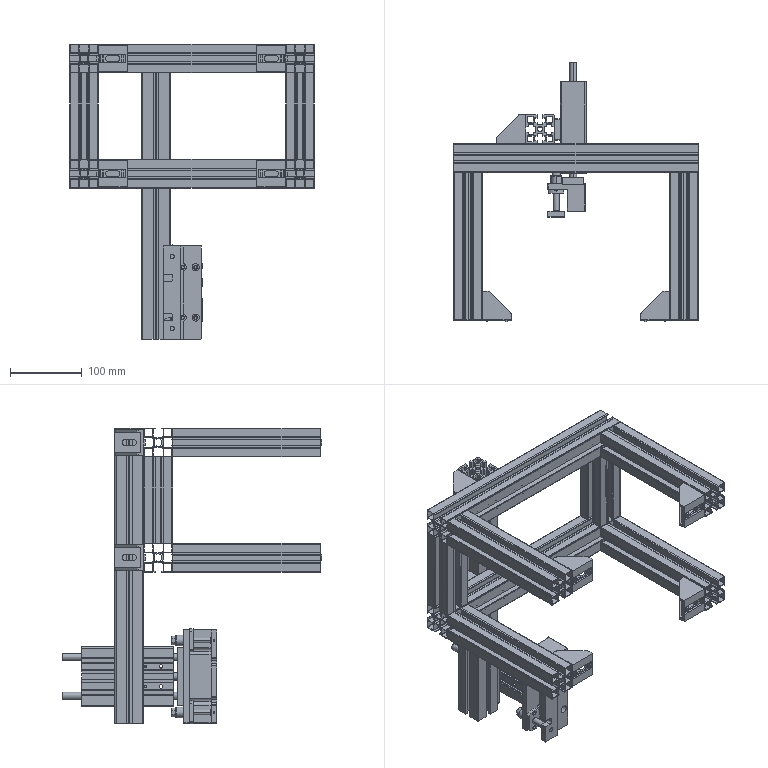Assembly | SolidWorks | mm | 17 component files | 24 solids | 1667 faces | box 340 x 360.1 x 411 mm | volume 1426037 mm3 | plane 1046 | cylinder 493 | cone 122 | spline 6 | commonest cylinder face diameters 4 x64 2.8 x48 6 x44 10.4 x40 2 x36 8.5 x28 3 x25 10 x20
Bill of materials:
4040-410AluminumProfile | 1 | A6061 | Long straight prismatic extrusion with a square cross-section. Each of the four sides has an open slot along its full length, there is a central round through-bore, and there are four hollow square cavities, one in each corner.
LH-CGJ-01-054 | 1 | A6061 | Flat rectangular strip with a round through-hole near each end. One long edge has two U-shaped notches with rounded ends, cut in from that edge and spaced apart along the length.
LH-CGJ-01-055 | 1 | A6061 | Rectangular bar or plate of moderate thickness. It has two larger round through-holes near the ends and two smaller holes in the middle, all on the centerline.
LH-CGJ-01-056 | 1 | SKD11 | Open rectangular frame built from several straight lengths of square slotted profile. Horizontal members form upper and lower rectangles or U-shapes, and vertical posts sit at the corners.
LH-CGJ-01-057 | 1 | Black POM | Rectangular block with a step at one end, giving an L-shaped profile. The large face has two large through-holes, several small holes, and two pairs of medium holes. Side holes and small edge notches are also visible.
LH-CGJ-01-058 | 2 | #45 | Stepped cylindrical pin: a short larger-diameter head, a long main shank, and a shorter reduced-diameter tip at the far end.
LME21-d8GuideBushing | 2 | SKD11 | Flanged bushing: a cylindrical boss projecting from a flat flange with two straight sides and two rounded ends. A central bore runs through, and there is a smaller mounting hole on each side of the bore.
NewG408-4040NationalStandardAngleCode | 2 | A6061 | Right-angle corner block, shaped like a solid gusset. Two flat outer faces sit at 90 degrees to each other. The profile has a triangular, chamfered top, and its corners are rounded. Each outer face has one through slot with rounded (obround) ends. Small raised rectangular tabs and narrow ribs stick out from the two outer faces next to the slots.
NewG408-4040NationalStandardAngleCode | 4 | A6061 | Triangular corner block with a diagonal outer face and rounded corners. The two perpendicular faces each have a long slot with rounded ends and small protruding locating tabs. Pockets and ribs are visible on the faces.
TCL-20x90-0_90fp | 1 | SKD11 | Rectangular end plate with three parallel round rods projecting from one face. The two outer rods are longer. The shorter middle rod ends in a larger-diameter cylindrical collar.
TC-L-20x9090_b | 1 | SKD11 | Rectangular extruded block. The long sides have lengthwise grooves and the end face has a notched outline. Three bores run along the length, the outer two open and the middle one apparently filled or plugged at the end. The side face has several counterbored cross holes.
Mates:
1. coincident | LH-CGJ-01-055-1 face at (-30.503, 90.215, 5.05) dir (1, 0, 0) | TCL20x90SCylinder-1/TC-L-20x9090_b-1 face at (-30.503, 171.215, 25.15) dir (-1, 0, 0)
2. width | TCL20x90SCylinder-1/TC-L-20x9090_b-1 face at (4.697, 171.215, 23.55) dir (0, 0, -1) | TCL20x90SCylinder-1/TC-L-20x9090_b-1 face at (-28.403, 171.215, 106.55) dir (0, 0, 1) | LH-CGJ-01-055-1 face at (-38.503, 90.215, 5.05) dir (0, 0, -1) | LH-CGJ-01-055-1 face at (-38.503, 90.215, 125.05) dir (0, 0, 1)
3. concentric | TCL20x90SCylinder-1/TC-L-20x9090_b-1 face at (-31.303, 105.215, 79.05) dir (1, 0, 0) r 2.75 | LH-CGJ-01-055-1 face at (-38.503, 105.215, 79.05) dir (-1, 0, 0) r 2.1
4. coincident | LH-CGJ-01-056-1 face at (-154.253, 85.215, 230.05) dir (0, 1, 0) | NewG408-4040NationalStandardAngleCode-1 face at (-78.503, 85.215, 212.05) dir (0, -1, 0)
5. width | LH-CGJ-01-057-1 face at (-29.503, 29.715, 130.05) dir (0, 0, 1) | LH-CGJ-01-057-1 face at (-29.503, 29.715, 0.05) dir (0, 0, -1) | TCL20x90SCylinder-1/TCL-20x90-0_90fp-1 face at (2.497, 38.215, 24.55) dir (0, 0, -1) | TCL20x90SCylinder-1/TCL-20x90-0_90fp-1 face at (-27.503, 38.215, 105.55) dir (0, 0, 1)
6. width | TCL20x90SCylinder-1/TCL-20x90-0_90fp-1 face at (2.497, 38.215, 105.55) dir (1, 0, 0) | TCL20x90SCylinder-1/TCL-20x90-0_90fp-1 face at (-27.503, 38.215, 24.55) dir (-1, 0, 0) | LH-CGJ-01-057-1 face at (-27.603, 29.715, 130.05) dir (1, 0, 0) | LH-CGJ-01-057-1 face at (2.597, 29.715, 130.05) dir (-1, 0, 0)
7. coincident | TCL20x90SCylinder-1/TCL-20x90-0_90fp-1 face at (-12.503, 28.215, 65.05) dir (0, -1, 0) | LH-CGJ-01-057-1 face at (2.597, 28.215, 130.05) dir (0, 1, 0)
8. concentric | LH-CGJ-01-057-1 face at (-36.003, 31.715, 15.05) dir (0, -1, 0) r 7.6 | LME21-d8GuideBushing-1 face at (-36.003, 16.715, 15.05) dir (0, 1, 0) r 7.5
9. parallel | LH-CGJ-01-057-1 face at (-47.503, 21.715, 0.05) dir (-1, 0, 0) | LME21-d8GuideBushing-1 face at (-46.503, 21.715, 2.977) dir (-1, 0, 0)
10. coincident | LH-CGJ-01-057-1 face at (-29.503, 21.715, 0.05) dir (0, -1, 0) | LME21-d8GuideBushing-1 face at (-36.003, 21.715, 15.05) dir (0, 1, 0)
11. concentric | LME21-d8GuideBushing-1 face at (-36.003, 16.715, 15.05) dir (0, 1, 0) r 4 | LH-CGJ-01-058-1 face at (-36.003, -16.285, 15.05) dir (0, -1, 0) r 4
12. coincident | LME21-d8GuideBushing-1 face at (-36.003, 40.715, 22.15) dir (0, 1, 0) | LH-CGJ-01-058-1 face at (-40.003, 40.715, 15.05) dir (0, -1, 0)
13. parallel | LH-CGJ-01-057-1 face at (-47.503, 21.715, 0.05) dir (-1, 0, 0) | LH-CGJ-01-058-1 face at (-41.503, 46.715, 17.448) dir (-1, 0, 0)
14. concentric | LH-CGJ-01-058-2 face at (-36.003, -16.285, 115.05) dir (0, -1, 0) r 3 | LH-CGJ-01-054-1 face at (-36.003, -8.285, 115.05) dir (0, 1, 0) r 3
15. concentric | LH-CGJ-01-058-1 face at (-36.003, -16.285, 15.05) dir (0, -1, 0) r 3 | LH-CGJ-01-054-1 face at (-36.003, -8.285, 15.05) dir (0, 1, 0) r 3
16. coincident | LH-CGJ-01-058-1 face at (-40.003, -8.285, 15.05) dir (0, -1, 0) | LH-CGJ-01-054-1 face at (-24.003, -8.285, 130.05) dir (0, 1, 0)
17. coincident | LH-CGJ-01-056-1 face at (-138.503, -159.885, 370.95) dir (1, 0, 0) | NewG408-4040NationalStandardAngleCode-3 face at (-138.503, -119.885, 407.95) dir (-1, 0, 0)
18. width | NewG408-4040NationalStandardAngleCode-3 face at (-101.503, -152.127, 407.95) dir (0, 0, 1) | NewG408-4040NationalStandardAngleCode-3 face at (-101.503, -152.127, 371.95) dir (0, 0, -1) | LH-CGJ-01-056-1 face at (-154.253, -159.885, 369.95) dir (0, 0, -1) | LH-CGJ-01-056-1 face at (-154.253, -159.885, 409.95) dir (0, 0, 1)
19. coincident | LH-CGJ-01-056-1 face at (-167.403, -159.885, 394.75) dir (0, -1, 0) | NewG408-4040NationalStandardAngleCode-3 face at (-138.503, -159.885, 407.95) dir (0, -1, 0)
20. coincident | LH-CGJ-01-056-1 face at (121.497, -159.885, 408.95) dir (-1, 0, 0) | NewG408-4040NationalStandardAngleCode-6 face at (121.497, -119.885, 371.95) dir (1, 0, 0)
21. coincident | NewG408-4040NationalStandardAngleCode-3 face at (-101.503, -152.127, 407.95) dir (0, 0, 1) | NewG408-4040NationalStandardAngleCode-6 face at (84.497, -152.127, 407.95) dir (0, 0, 1)
22. coincident | NewG408-4040NationalStandardAngleCode-3 face at (-138.503, -159.885, 407.95) dir (0, -1, 0) | NewG408-4040NationalStandardAngleCode-6 face at (121.497, -159.885, 371.95) dir (0, -1, 0)
23. width | NewG408-4040NationalStandardAngleCode-1 face at (-115.503, 92.973, 212.05) dir (0, 0, -1) | NewG408-4040NationalStandardAngleCode-1 face at (-115.503, 92.973, 248.05) dir (0, 0, 1) | LH-CGJ-01-056-1 face at (141.497, 84.215, 250.05) dir (0, 0, 1) | LH-CGJ-01-056-1 face at (141.497, 84.215, 210.05) dir (0, 0, -1)
24. coincident | 4040-410AluminumProfile-1 face at (-38.503, 123.715, 0.05) dir (1, 0, 0) | LH-CGJ-01-055-1 face at (-38.503, 90.215, 5.05) dir (-1, 0, 0)
25. width | 4040-410AluminumProfile-1 face at (-54.353, 125.215, 0.05) dir (0, 1, 0) | 4040-410AluminumProfile-1 face at (-40.003, 85.215, 0.05) dir (0, -1, 0) | LH-CGJ-01-055-1 face at (-38.503, 90.215, 5.05) dir (0, -1, 0) | LH-CGJ-01-055-1 face at (-38.503, 120.215, 5.05) dir (0, 1, 0)
26. distance | 4040-410AluminumProfile-1 face at (-77.003, 86.715, 0.05) dir (0, 0, -1) | LH-CGJ-01-055-1 face at (-38.503, 90.215, 5.05) dir (0, 0, -1)
27. coincident | LH-CGJ-01-056-1 face at (141.497, 85.215, 225.8) dir (0, 1, 0) | 4040-410AluminumProfile-1 face at (-40.003, 85.215, 0.05) dir (0, -1, 0)
28. coincident | LH-CGJ-01-056-1 face at (-158.503, 84.215, 410.05) dir (0, 0, 1) | 4040-410AluminumProfile-1 face at (-77.003, 86.715, 410.05) dir (0, 0, 1)
29. distance | 4040-410AluminumProfile-1 face at (-78.503, 86.715, 0.05) dir (-1, 0, 0) | LH-CGJ-01-056-1 face at (-178.503, 84.215, 230.05) dir (-1, 0, 0)
30. coincident | LH-CGJ-01-056-1 face at (-158.503, 84.215, 410.05) dir (0, 0, 1) | 4040-410AluminumProfile-1 face at (-77.003, 86.715, 410.05) dir (0, 0, 1)
31. concentric | TC-L-20x9090_b-1 face at (127, 27, 0) dir (-1, 0, 0) r 8.5 | TCL-20x90-0_90fp-1 face at (154, 27, 0) dir (-1, 0, 0) r 5
32. concentric | TC-L-20x9090_b-1 face at (127, -27, 0) dir (-1, 0, 0) r 8.5 | TCL-20x90-0_90fp-1 face at (154, -27, 0) dir (-1, 0, 0) r 5
33. distance | TC-L-20x9090_b-1 face at (0, -24.9, -15.4) dir (-1, 0, 0) | TCL-20x90-0_90fp-1 face at (-6, 0, 0) dir (1, 0, 0)